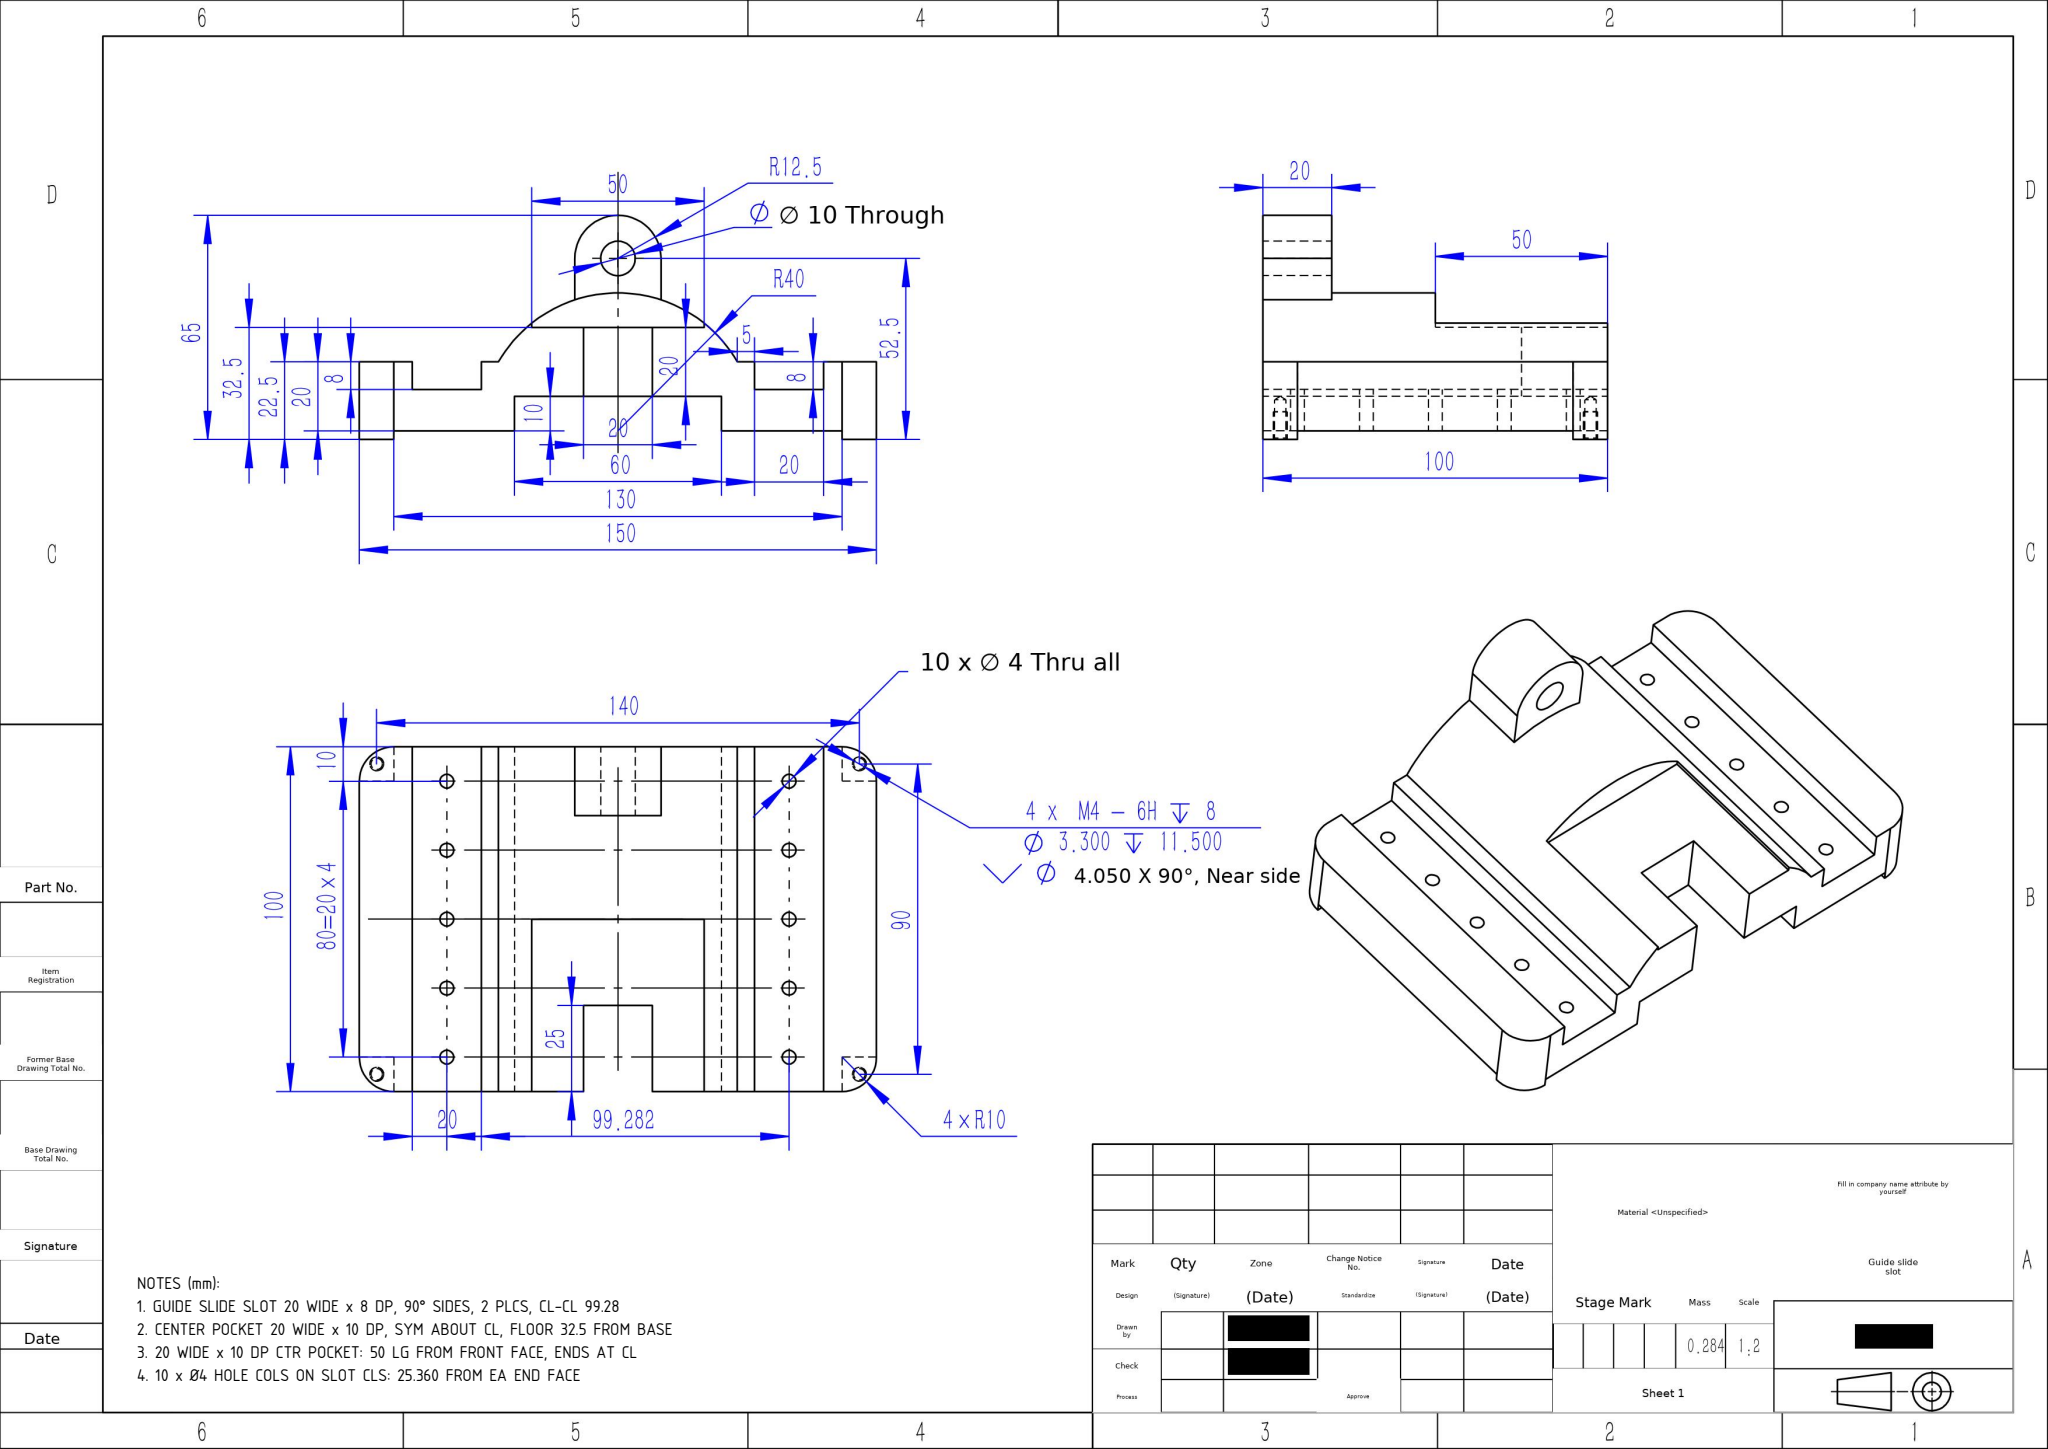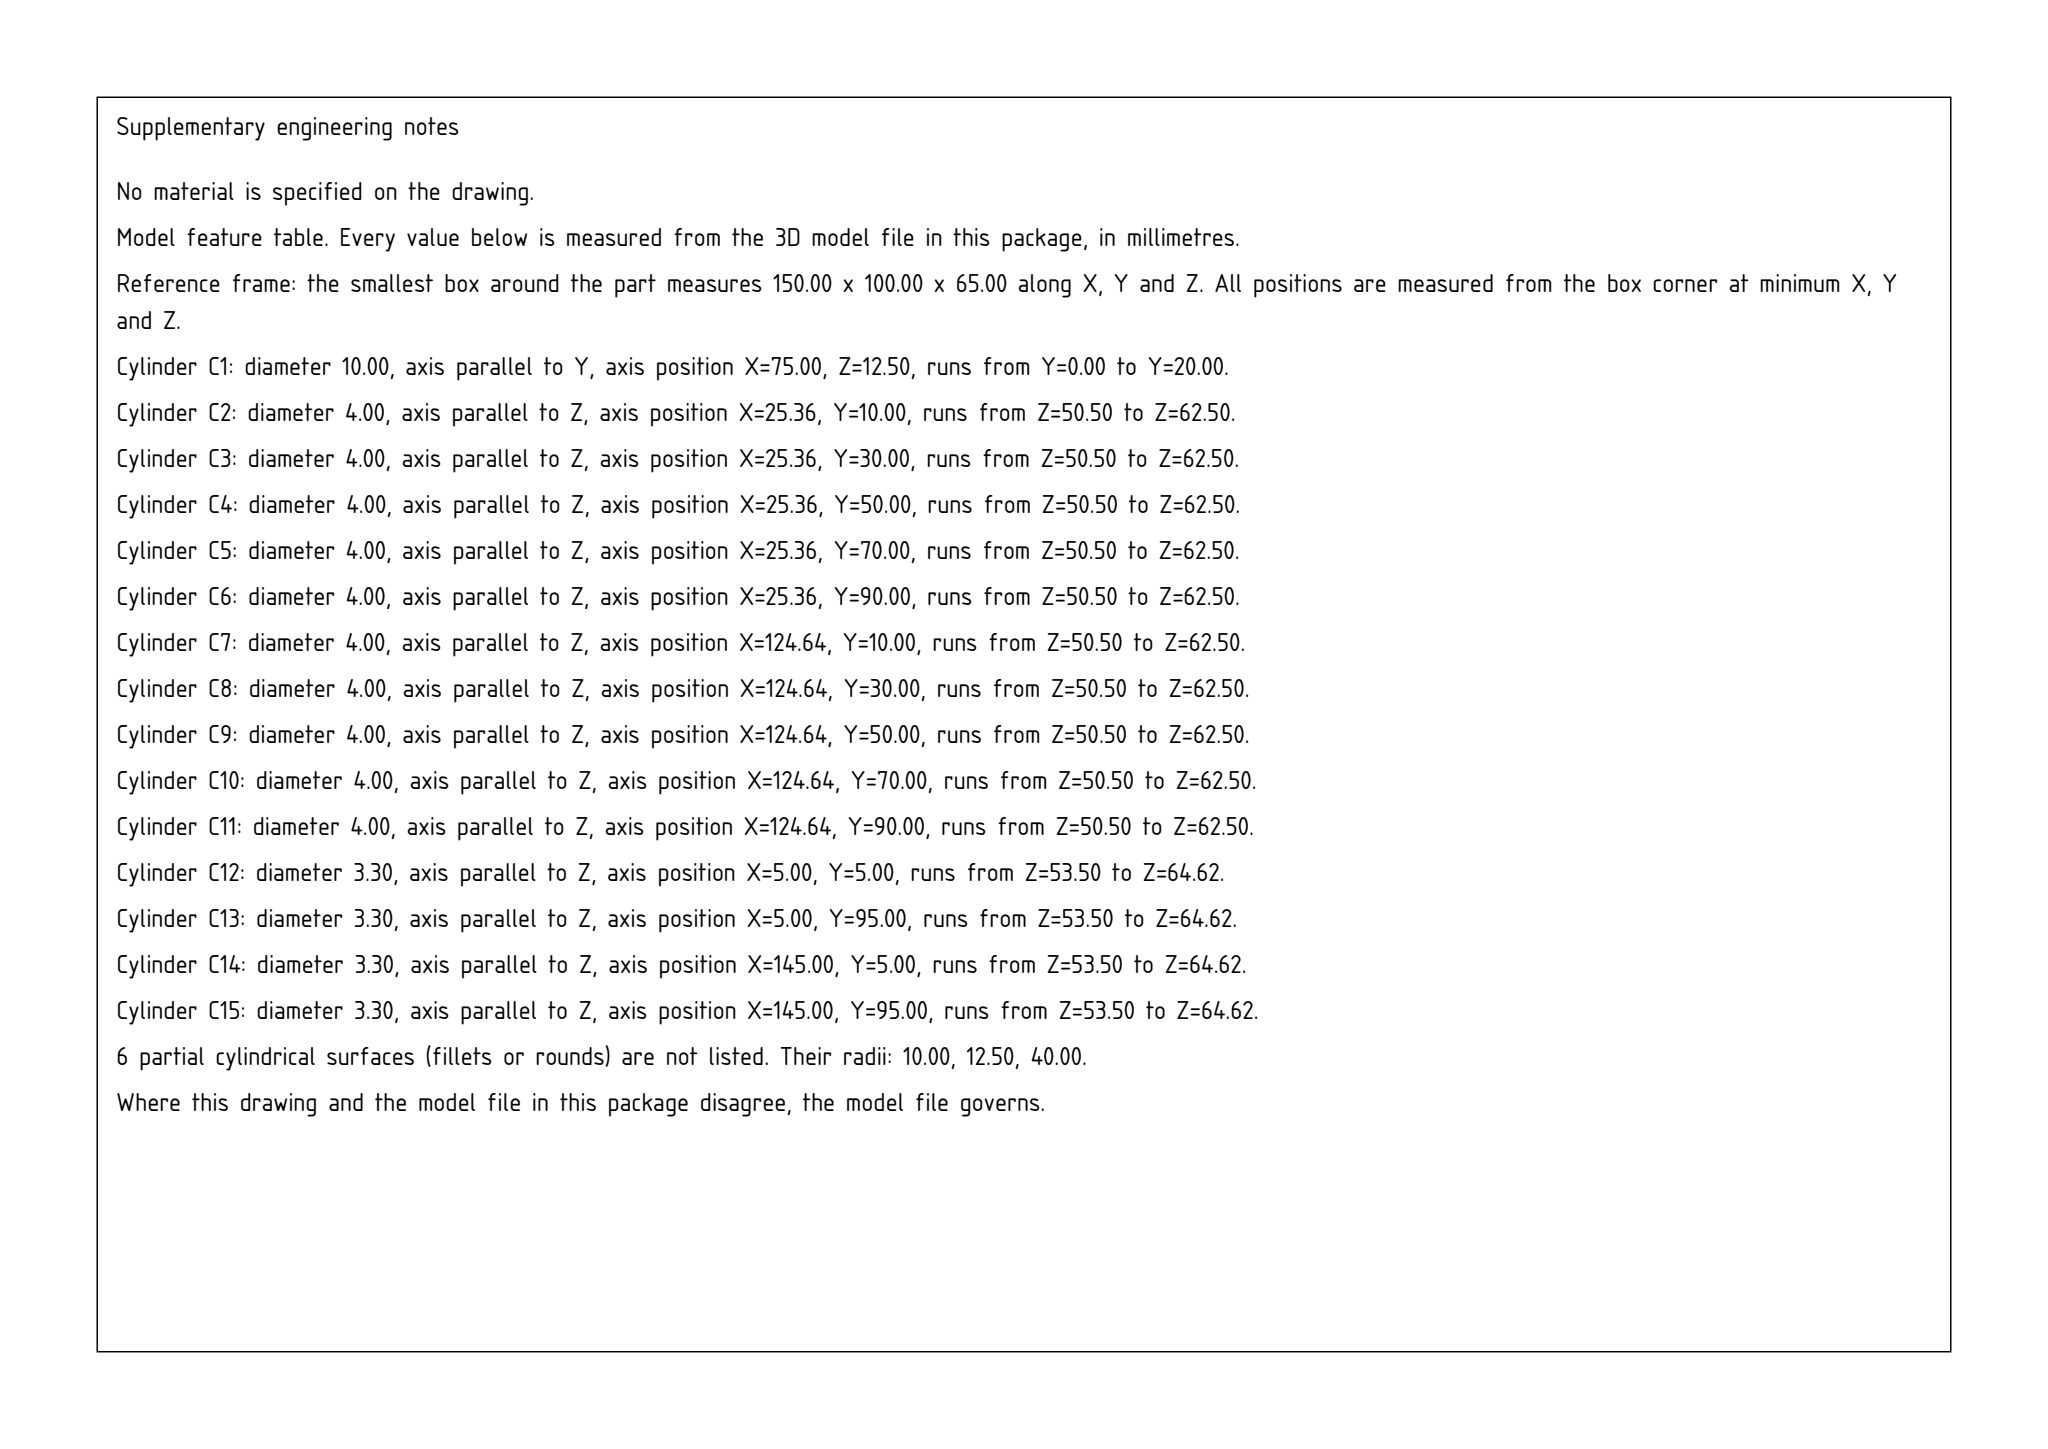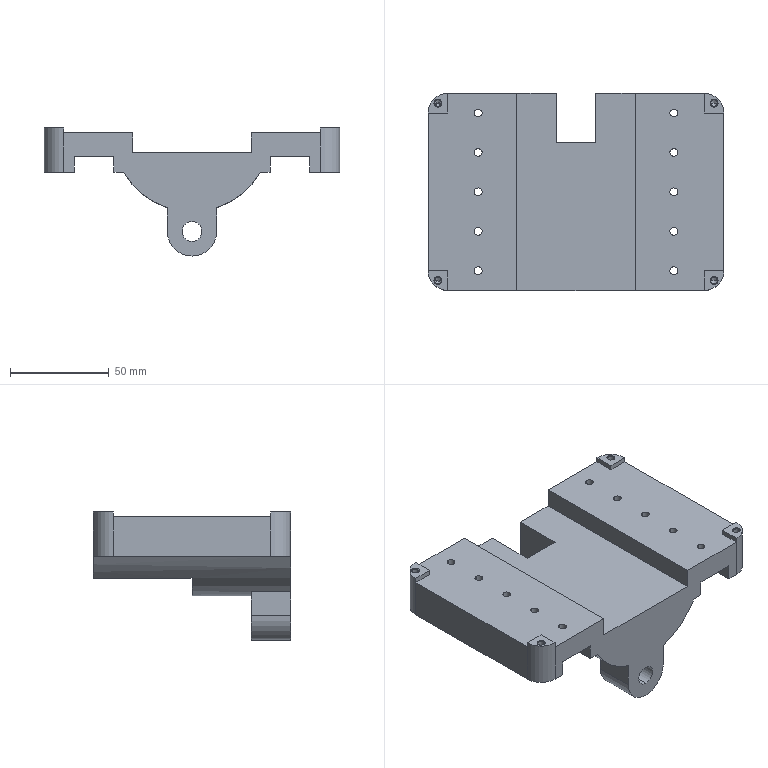Part | SolidWorks | mm | 1 solid | 96 faces | box 150 x 100 x 65 mm | volume 284049 mm3 | plane 42 | cylinder 38 | cone 16 | commonest cylinder face diameters 4 x20 3.3 x8 20 x4 10 x2 25 x2 80 x2
Drawing notes:
GUIDE SLIDE SLOT 20 WIDE x 8 DP, 90° SIDES, 2 PLCS, CL-CL 99.28 | from the solid: X planes 15.36/35.36 and 114.64/134.64 give 20 wide, axis-normal walls = 90°; slot floor z=50.5 vs rail face z=42.5 = 8 DP; slot CLs x=25.36 & 124.64 = 99.28 apart
CENTER POCKET 20 WIDE x 10 DP, SYM ABOUT CL, FLOOR 32.5 FROM BASE | from the solid: X planes 65.0 and 85.0 = 20 wide, sym about part CL x=75; floor plane z=32.5, 10 below z=42.5 face; pocket end plane y=75
20 WIDE x 10 DP CTR POCKET: 50 LG FROM FRONT FACE, ENDS AT CL | from the solid: x planes 65 & 85 (20 wide, sym abt x=75); unique y plane at 50 with pocket open at y=0 -> 50 long ending at part CL (100/2)
10 x Ø4 HOLE COLS ON SLOT CLS: 25.360 FROM EA END FACE | from the solid: Ø4 z-axis holes at x=25.36 and x=124.64; 150-124.64=25.36; CL-CL=99.282